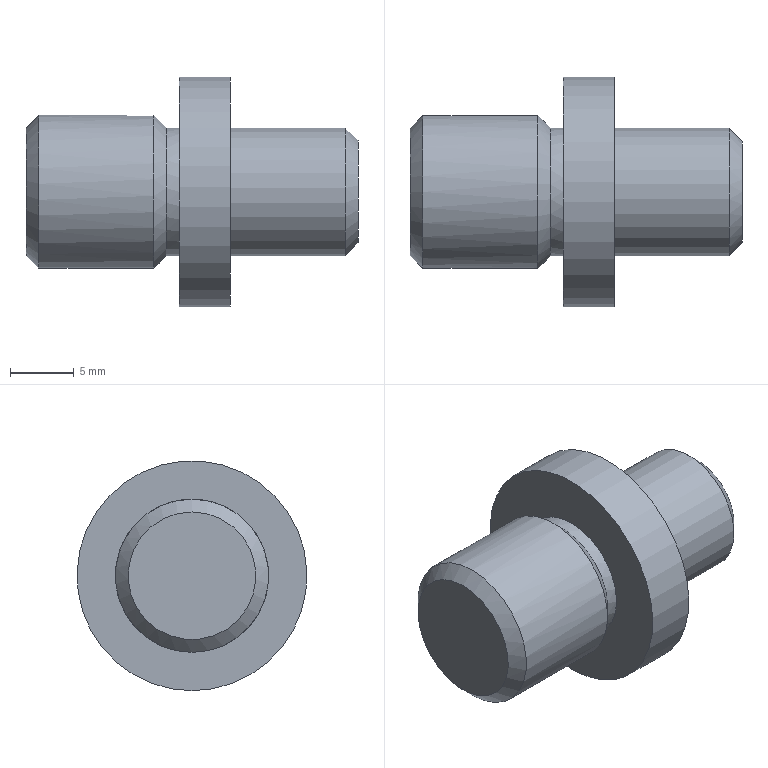Component | NX | A_LOCATING_PIN | 1 solid | 11 faces | box 26 x 18 x 18 mm | volume 3076 mm3 | plane 4 | cylinder 4 | cone 3 | commonest cylinder face diameters 10 x2 12 x1 18 x1
STEP:
#1=CARTESIAN_POINT('',(0.,0.,0.));
#2=DIRECTION('',(0.,0.,1.));
#3=DIRECTION('',(1.,0.,0.));
#4=AXIS2_PLACEMENT_3D('',#1,#2,#3);
#5=CARTESIAN_POINT('',(-41.,13.9,-11.5));
#6=VERTEX_POINT('',#5);
#7=CARTESIAN_POINT('',(-41.,13.9,-16.5));
#8=DIRECTION('',(-1.,0.,0.));
#9=DIRECTION('',(0.,0.,1.));
#10=AXIS2_PLACEMENT_3D('',#7,#8,#9);
#11=CIRCLE('',#10,5.);
#12=CARTESIAN_POINT('',(-41.,13.9,-16.5));
#13=DIRECTION('',(-1.,0.,0.));
#14=DIRECTION('',(0.,0.,1.));
#15=AXIS2_PLACEMENT_3D('',#12,#13,#14);
#16=PLANE('',#15);
#17=CARTESIAN_POINT('',(0.,0.));
#18=DIRECTION('',(1.,0.));
#19=AXIS2_PLACEMENT_2D('',#17,#18);
#20=CIRCLE('',#19,5.);
#21=(GEOMETRIC_REPRESENTATION_CONTEXT(2)PARAMETRIC_REPRESENTATION_CONTEXT()REPRESENTATION_CONTEXT('',''));
#22=DEFINITIONAL_REPRESENTATION('',(#20),#21);
#23=PCURVE('',#16,#22);
#24=CARTESIAN_POINT('',(-40.,13.9,-16.5));
#25=DIRECTION('',(1.,0.,0.));
#26=DIRECTION('',(0.,0.,-1.));
#27=AXIS2_PLACEMENT_3D('',#24,#25,#26);
#28=CONICAL_SURFACE('',#27,6.,0.7854);
#29=CARTESIAN_POINT('',(9.425,-1.));
#30=DIRECTION('',(-1.,0.));
#31=VECTOR('',#30,1.);
#32=LINE('',#29,#31);
#33=(GEOMETRIC_REPRESENTATION_CONTEXT(2)PARAMETRIC_REPRESENTATION_CONTEXT()REPRESENTATION_CONTEXT('',''));
#34=DEFINITIONAL_REPRESENTATION('',(#32),#33);
#35=PCURVE('',#28,#34);
#36=SURFACE_CURVE('',#11,(#23,#35),.PCURVE_S1.);
#37=EDGE_CURVE('',#6,#6,#36,.T.);
#38=ORIENTED_EDGE('',*,*,#37,.T.);
#39=EDGE_LOOP('',(#38));
#40=FACE_BOUND('',#39,.T.);
#41=ADVANCED_FACE('',(#40),#16,.T.);
#42=CARTESIAN_POINT('',(-31.,13.9,-22.5));
#43=VERTEX_POINT('',#42);
#44=CARTESIAN_POINT('',(-31.,13.9,-16.5));
#45=DIRECTION('',(-1.,0.,0.));
#46=DIRECTION('',(0.,0.,-1.));
#47=AXIS2_PLACEMENT_3D('',#44,#45,#46);
#48=CIRCLE('',#47,6.);
#49=CARTESIAN_POINT('',(-41.,13.9,-16.5));
#50=DIRECTION('',(1.,0.,0.));
#51=DIRECTION('',(0.,0.,-1.));
#52=AXIS2_PLACEMENT_3D('',#49,#50,#51);
#53=CYLINDRICAL_SURFACE('',#52,6.);
#54=CARTESIAN_POINT('',(6.283,10.));
#55=DIRECTION('',(-1.,0.));
#56=VECTOR('',#55,1.);
#57=LINE('',#54,#56);
#58=(GEOMETRIC_REPRESENTATION_CONTEXT(2)PARAMETRIC_REPRESENTATION_CONTEXT()REPRESENTATION_CONTEXT('',''));
#59=DEFINITIONAL_REPRESENTATION('',(#57),#58);
#60=PCURVE('',#53,#59);
#61=CARTESIAN_POINT('',(-31.,13.9,-16.5));
#62=DIRECTION('',(-1.,0.,0.));
#63=DIRECTION('',(0.,0.,1.));
#64=AXIS2_PLACEMENT_3D('',#61,#62,#63);
#65=CONICAL_SURFACE('',#64,6.,0.7854);
#66=CARTESIAN_POINT('',(3.142,0.));
#67=DIRECTION('',(1.,0.));
#68=VECTOR('',#67,1.);
#69=LINE('',#66,#68);
#70=(GEOMETRIC_REPRESENTATION_CONTEXT(2)PARAMETRIC_REPRESENTATION_CONTEXT()REPRESENTATION_CONTEXT('',''));
#71=DEFINITIONAL_REPRESENTATION('',(#69),#70);
#72=PCURVE('',#65,#71);
#73=SURFACE_CURVE('',#48,(#60,#72),.PCURVE_S1.);
#74=EDGE_CURVE('',#43,#43,#73,.T.);
#75=ORIENTED_EDGE('',*,*,#74,.T.);
#76=CARTESIAN_POINT('',(-40.,13.9,-22.5));
#77=VERTEX_POINT('',#76);
#78=CARTESIAN_POINT('',(-40.,13.9,-22.5));
#79=CARTESIAN_POINT('',(-31.,13.9,-22.5));
#80=B_SPLINE_CURVE_WITH_KNOTS('',1,(#78,#79),.UNSPECIFIED.,.F.,.F.,(2,2),(1.,10.),.PIECEWISE_BEZIER_KNOTS.);
#81=CARTESIAN_POINT('',(0.,0.));
#82=DIRECTION('',(0.,1.));
#83=VECTOR('',#82,1.);
#84=LINE('',#81,#83);
#85=(GEOMETRIC_REPRESENTATION_CONTEXT(2)PARAMETRIC_REPRESENTATION_CONTEXT()REPRESENTATION_CONTEXT('',''));
#86=DEFINITIONAL_REPRESENTATION('',(#84),#85);
#87=PCURVE('',#53,#86);
#88=CARTESIAN_POINT('',(6.283,0.));
#89=DIRECTION('',(0.,1.));
#90=VECTOR('',#89,1.);
#91=LINE('',#88,#90);
#92=(GEOMETRIC_REPRESENTATION_CONTEXT(2)PARAMETRIC_REPRESENTATION_CONTEXT()REPRESENTATION_CONTEXT('',''));
#93=DEFINITIONAL_REPRESENTATION('',(#91),#92);
#94=PCURVE('',#53,#93);
#95=SEAM_CURVE('',#80,(#87,#94),.PCURVE_S1.);
#96=EDGE_CURVE('',#77,#43,#95,.T.);
#97=ORIENTED_EDGE('',*,*,#96,.F.);
#98=CARTESIAN_POINT('',(-40.,13.9,-10.5));
#99=VERTEX_POINT('',#98);
#100=CARTESIAN_POINT('',(-40.,13.9,-16.5));
#101=DIRECTION('',(1.,0.,0.));
#102=DIRECTION('',(0.,0.,1.));
#103=AXIS2_PLACEMENT_3D('',#100,#101,#102);
#104=CIRCLE('',#103,6.);
#105=CARTESIAN_POINT('',(-3.142,1.));
#106=DIRECTION('',(1.,0.));
#107=VECTOR('',#106,1.);
#108=LINE('',#105,#107);
#109=(GEOMETRIC_REPRESENTATION_CONTEXT(2)PARAMETRIC_REPRESENTATION_CONTEXT()REPRESENTATION_CONTEXT('',''));
#110=DEFINITIONAL_REPRESENTATION('',(#108),#109);
#111=PCURVE('',#53,#110);
#112=CARTESIAN_POINT('',(3.142,0.));
#113=DIRECTION('',(1.,0.));
#114=VECTOR('',#113,1.);
#115=LINE('',#112,#114);
#116=(GEOMETRIC_REPRESENTATION_CONTEXT(2)PARAMETRIC_REPRESENTATION_CONTEXT()REPRESENTATION_CONTEXT('',''));
#117=DEFINITIONAL_REPRESENTATION('',(#115),#116);
#118=PCURVE('',#28,#117);
#119=SURFACE_CURVE('',#104,(#111,#118),.PCURVE_S1.);
#120=EDGE_CURVE('',#77,#99,#119,.T.);
#121=ORIENTED_EDGE('',*,*,#120,.T.);
#122=CARTESIAN_POINT('',(-40.,13.9,-16.5));
#123=DIRECTION('',(1.,0.,0.));
#124=DIRECTION('',(0.,0.,1.));
#125=AXIS2_PLACEMENT_3D('',#122,#123,#124);
#126=CIRCLE('',#125,6.);
#127=CARTESIAN_POINT('',(3.142,1.));
#128=DIRECTION('',(1.,0.));
#129=VECTOR('',#128,1.);
#130=LINE('',#127,#129);
#131=(GEOMETRIC_REPRESENTATION_CONTEXT(2)PARAMETRIC_REPRESENTATION_CONTEXT()REPRESENTATION_CONTEXT('',''));
#132=DEFINITIONAL_REPRESENTATION('',(#130),#131);
#133=PCURVE('',#53,#132);
#134=CARTESIAN_POINT('',(3.142,0.));
#135=DIRECTION('',(1.,0.));
#136=VECTOR('',#135,1.);
#137=LINE('',#134,#136);
#138=(GEOMETRIC_REPRESENTATION_CONTEXT(2)PARAMETRIC_REPRESENTATION_CONTEXT()REPRESENTATION_CONTEXT('',''));
#139=DEFINITIONAL_REPRESENTATION('',(#137),#138);
#140=PCURVE('',#28,#139);
#141=SURFACE_CURVE('',#126,(#133,#140),.PCURVE_S1.);
#142=EDGE_CURVE('',#99,#77,#141,.T.);
#143=ORIENTED_EDGE('',*,*,#142,.T.);
#144=ORIENTED_EDGE('',*,*,#96,.T.);
#145=EDGE_LOOP('',(#75,#97,#121,#143,#144));
#146=FACE_BOUND('',#145,.T.);
#147=ADVANCED_FACE('',(#146),#53,.T.);
#148=CARTESIAN_POINT('',(-29.,13.9,-21.5));
#149=VERTEX_POINT('',#148);
#150=CARTESIAN_POINT('',(-29.,13.9,-11.5));
#151=VERTEX_POINT('',#150);
#152=CARTESIAN_POINT('',(-29.,13.9,-16.5));
#153=DIRECTION('',(1.,0.,0.));
#154=DIRECTION('',(0.,0.,1.));
#155=AXIS2_PLACEMENT_3D('',#152,#153,#154);
#156=CIRCLE('',#155,5.);
#157=CARTESIAN_POINT('',(-30.,13.9,-16.5));
#158=DIRECTION('',(1.,0.,0.));
#159=DIRECTION('',(0.,0.,-1.));
#160=AXIS2_PLACEMENT_3D('',#157,#158,#159);
#161=CYLINDRICAL_SURFACE('',#160,5.);
#162=CARTESIAN_POINT('',(-3.142,1.));
#163=DIRECTION('',(1.,0.));
#164=VECTOR('',#163,1.);
#165=LINE('',#162,#164);
#166=(GEOMETRIC_REPRESENTATION_CONTEXT(2)PARAMETRIC_REPRESENTATION_CONTEXT()REPRESENTATION_CONTEXT('',''));
#167=DEFINITIONAL_REPRESENTATION('',(#165),#166);
#168=PCURVE('',#161,#167);
#169=CARTESIAN_POINT('',(-29.,13.9,-16.5));
#170=DIRECTION('',(-1.,0.,0.));
#171=DIRECTION('',(0.,0.,1.));
#172=AXIS2_PLACEMENT_3D('',#169,#170,#171);
#173=PLANE('',#172);
#174=CARTESIAN_POINT('',(5.,0.));
#175=CARTESIAN_POINT('',(5.,-8.66));
#176=CARTESIAN_POINT('',(-2.5,-4.33));
#177=CARTESIAN_POINT('',(-10.,-0.));
#178=CARTESIAN_POINT('',(-2.5,4.33));
#179=CARTESIAN_POINT('',(5.,8.66));
#180=CARTESIAN_POINT('',(5.,0.));
#181=(BOUNDED_CURVE()B_SPLINE_CURVE(2,(#174,#175,#176,#177,#178,#179,#180),.UNSPECIFIED.,.T.,.F.)B_SPLINE_CURVE_WITH_KNOTS((1,2,2,2,2,1),(-2.094,0.,2.094,4.189,6.283,8.378),.UNSPECIFIED.)CURVE()GEOMETRIC_REPRESENTATION_ITEM()RATIONAL_B_SPLINE_CURVE((1.,0.5,1.,0.5,1.,0.5,1.))REPRESENTATION_ITEM(''));
#182=(GEOMETRIC_REPRESENTATION_CONTEXT(2)PARAMETRIC_REPRESENTATION_CONTEXT()REPRESENTATION_CONTEXT('',''));
#183=DEFINITIONAL_REPRESENTATION('',(#181),#182);
#184=PCURVE('',#173,#183);
#185=SURFACE_CURVE('',#156,(#168,#184),.PCURVE_S1.);
#186=EDGE_CURVE('',#149,#151,#185,.T.);
#187=ORIENTED_EDGE('',*,*,#186,.F.);
#188=CARTESIAN_POINT('',(-30.,13.9,-21.5));
#189=VERTEX_POINT('',#188);
#190=CARTESIAN_POINT('',(-30.,13.9,-21.5));
#191=CARTESIAN_POINT('',(-29.,13.9,-21.5));
#192=B_SPLINE_CURVE_WITH_KNOTS('',1,(#190,#191),.UNSPECIFIED.,.F.,.F.,(2,2),(0.,1.),.PIECEWISE_BEZIER_KNOTS.);
#193=CARTESIAN_POINT('',(0.,0.));
#194=DIRECTION('',(0.,1.));
#195=VECTOR('',#194,1.);
#196=LINE('',#193,#195);
#197=(GEOMETRIC_REPRESENTATION_CONTEXT(2)PARAMETRIC_REPRESENTATION_CONTEXT()REPRESENTATION_CONTEXT('',''));
#198=DEFINITIONAL_REPRESENTATION('',(#196),#197);
#199=PCURVE('',#161,#198);
#200=CARTESIAN_POINT('',(6.283,0.));
#201=DIRECTION('',(0.,1.));
#202=VECTOR('',#201,1.);
#203=LINE('',#200,#202);
#204=(GEOMETRIC_REPRESENTATION_CONTEXT(2)PARAMETRIC_REPRESENTATION_CONTEXT()REPRESENTATION_CONTEXT('',''));
#205=DEFINITIONAL_REPRESENTATION('',(#203),#204);
#206=PCURVE('',#161,#205);
#207=SEAM_CURVE('',#192,(#199,#206),.PCURVE_S1.);
#208=EDGE_CURVE('',#189,#149,#207,.T.);
#209=ORIENTED_EDGE('',*,*,#208,.F.);
#210=CARTESIAN_POINT('',(-30.,13.9,-16.5));
#211=DIRECTION('',(1.,0.,0.));
#212=DIRECTION('',(0.,0.,-1.));
#213=AXIS2_PLACEMENT_3D('',#210,#211,#212);
#214=CIRCLE('',#213,5.);
#215=CARTESIAN_POINT('',(0.,0.));
#216=DIRECTION('',(1.,0.));
#217=VECTOR('',#216,1.);
#218=LINE('',#215,#217);
#219=(GEOMETRIC_REPRESENTATION_CONTEXT(2)PARAMETRIC_REPRESENTATION_CONTEXT()REPRESENTATION_CONTEXT('',''));
#220=DEFINITIONAL_REPRESENTATION('',(#218),#219);
#221=PCURVE('',#161,#220);
#222=CARTESIAN_POINT('',(9.425,-1.));
#223=DIRECTION('',(-1.,0.));
#224=VECTOR('',#223,1.);
#225=LINE('',#222,#224);
#226=(GEOMETRIC_REPRESENTATION_CONTEXT(2)PARAMETRIC_REPRESENTATION_CONTEXT()REPRESENTATION_CONTEXT('',''));
#227=DEFINITIONAL_REPRESENTATION('',(#225),#226);
#228=PCURVE('',#65,#227);
#229=SURFACE_CURVE('',#214,(#221,#228),.PCURVE_S1.);
#230=EDGE_CURVE('',#189,#189,#229,.T.);
#231=ORIENTED_EDGE('',*,*,#230,.T.);
#232=ORIENTED_EDGE('',*,*,#208,.T.);
#233=CARTESIAN_POINT('',(-29.,13.9,-16.5));
#234=DIRECTION('',(1.,0.,0.));
#235=DIRECTION('',(0.,0.,1.));
#236=AXIS2_PLACEMENT_3D('',#233,#234,#235);
#237=CIRCLE('',#236,5.);
#238=CARTESIAN_POINT('',(3.142,1.));
#239=DIRECTION('',(1.,0.));
#240=VECTOR('',#239,1.);
#241=LINE('',#238,#240);
#242=(GEOMETRIC_REPRESENTATION_CONTEXT(2)PARAMETRIC_REPRESENTATION_CONTEXT()REPRESENTATION_CONTEXT('',''));
#243=DEFINITIONAL_REPRESENTATION('',(#241),#242);
#244=PCURVE('',#161,#243);
#245=CARTESIAN_POINT('',(5.,0.));
#246=CARTESIAN_POINT('',(5.,-8.66));
#247=CARTESIAN_POINT('',(-2.5,-4.33));
#248=CARTESIAN_POINT('',(-10.,-0.));
#249=CARTESIAN_POINT('',(-2.5,4.33));
#250=CARTESIAN_POINT('',(5.,8.66));
#251=CARTESIAN_POINT('',(5.,0.));
#252=(BOUNDED_CURVE()B_SPLINE_CURVE(2,(#245,#246,#247,#248,#249,#250,#251),.UNSPECIFIED.,.T.,.F.)B_SPLINE_CURVE_WITH_KNOTS((1,2,2,2,2,1),(-2.094,0.,2.094,4.189,6.283,8.378),.UNSPECIFIED.)CURVE()GEOMETRIC_REPRESENTATION_ITEM()RATIONAL_B_SPLINE_CURVE((1.,0.5,1.,0.5,1.,0.5,1.))REPRESENTATION_ITEM(''));
#253=(GEOMETRIC_REPRESENTATION_CONTEXT(2)PARAMETRIC_REPRESENTATION_CONTEXT()REPRESENTATION_CONTEXT('',''));
#254=DEFINITIONAL_REPRESENTATION('',(#252),#253);
#255=PCURVE('',#173,#254);
#256=SURFACE_CURVE('',#237,(#244,#255),.PCURVE_S1.);
#257=EDGE_CURVE('',#151,#149,#256,.T.);
#258=ORIENTED_EDGE('',*,*,#257,.F.);
#259=EDGE_LOOP('',(#187,#209,#231,#232,#258));
#260=FACE_BOUND('',#259,.T.);
#261=ADVANCED_FACE('',(#260),#161,.T.);
#262=CARTESIAN_POINT('',(-25.,13.9,-21.5));
#263=VERTEX_POINT('',#262);
#264=CARTESIAN_POINT('',(-25.,13.9,-16.5));
#265=DIRECTION('',(1.,0.,0.));
#266=DIRECTION('',(0.,0.,-1.));
#267=AXIS2_PLACEMENT_3D('',#264,#265,#266);
#268=CIRCLE('',#267,5.);
#269=CARTESIAN_POINT('',(-25.,13.9,-16.5));
#270=DIRECTION('',(1.,0.,0.));
#271=DIRECTION('',(0.,0.,-1.));
#272=AXIS2_PLACEMENT_3D('',#269,#270,#271);
#273=PLANE('',#272);
#274=CARTESIAN_POINT('',(0.,0.));
#275=DIRECTION('',(1.,0.));
#276=AXIS2_PLACEMENT_2D('',#274,#275);
#277=CIRCLE('',#276,5.);
#278=(GEOMETRIC_REPRESENTATION_CONTEXT(2)PARAMETRIC_REPRESENTATION_CONTEXT()REPRESENTATION_CONTEXT('',''));
#279=DEFINITIONAL_REPRESENTATION('',(#277),#278);
#280=PCURVE('',#273,#279);
#281=CARTESIAN_POINT('',(-25.,13.9,-16.5));
#282=DIRECTION('',(1.,0.,0.));
#283=DIRECTION('',(0.,0.,-1.));
#284=AXIS2_PLACEMENT_3D('',#281,#282,#283);
#285=CYLINDRICAL_SURFACE('',#284,5.);
#286=CARTESIAN_POINT('',(0.,0.));
#287=DIRECTION('',(1.,0.));
#288=VECTOR('',#287,1.);
#289=LINE('',#286,#288);
#290=(GEOMETRIC_REPRESENTATION_CONTEXT(2)PARAMETRIC_REPRESENTATION_CONTEXT()REPRESENTATION_CONTEXT('',''));
#291=DEFINITIONAL_REPRESENTATION('',(#289),#290);
#292=PCURVE('',#285,#291);
#293=SURFACE_CURVE('',#268,(#280,#292),.PCURVE_S1.);
#294=EDGE_CURVE('',#263,#263,#293,.T.);
#295=ORIENTED_EDGE('',*,*,#294,.F.);
#296=EDGE_LOOP('',(#295));
#297=FACE_BOUND('',#296,.T.);
#298=CARTESIAN_POINT('',(-25.,13.9,-25.5));
#299=VERTEX_POINT('',#298);
#300=CARTESIAN_POINT('',(-25.,13.9,-16.5));
#301=DIRECTION('',(-1.,0.,0.));
#302=DIRECTION('',(0.,0.,-1.));
#303=AXIS2_PLACEMENT_3D('',#300,#301,#302);
#304=CIRCLE('',#303,9.);
#305=CARTESIAN_POINT('',(9.,0.));
#306=CARTESIAN_POINT('',(9.,-15.588));
#307=CARTESIAN_POINT('',(-4.5,-7.794));
#308=CARTESIAN_POINT('',(-18.,-0.));
#309=CARTESIAN_POINT('',(-4.5,7.794));
#310=CARTESIAN_POINT('',(9.,15.588));
#311=CARTESIAN_POINT('',(9.,0.));
#312=(BOUNDED_CURVE()B_SPLINE_CURVE(2,(#305,#306,#307,#308,#309,#310,#311),.UNSPECIFIED.,.T.,.F.)B_SPLINE_CURVE_WITH_KNOTS((1,2,2,2,2,1),(-2.094,0.,2.094,4.189,6.283,8.378),.UNSPECIFIED.)CURVE()GEOMETRIC_REPRESENTATION_ITEM()RATIONAL_B_SPLINE_CURVE((1.,0.5,1.,0.5,1.,0.5,1.))REPRESENTATION_ITEM(''));
#313=(GEOMETRIC_REPRESENTATION_CONTEXT(2)PARAMETRIC_REPRESENTATION_CONTEXT()REPRESENTATION_CONTEXT('',''));
#314=DEFINITIONAL_REPRESENTATION('',(#312),#313);
#315=PCURVE('',#273,#314);
#316=CARTESIAN_POINT('',(-29.,13.9,-16.5));
#317=DIRECTION('',(1.,0.,0.));
#318=DIRECTION('',(0.,0.,-1.));
#319=AXIS2_PLACEMENT_3D('',#316,#317,#318);
#320=CYLINDRICAL_SURFACE('',#319,9.);
#321=CARTESIAN_POINT('',(6.283,4.));
#322=DIRECTION('',(-1.,0.));
#323=VECTOR('',#322,1.);
#324=LINE('',#321,#323);
#325=(GEOMETRIC_REPRESENTATION_CONTEXT(2)PARAMETRIC_REPRESENTATION_CONTEXT()REPRESENTATION_CONTEXT('',''));
#326=DEFINITIONAL_REPRESENTATION('',(#324),#325);
#327=PCURVE('',#320,#326);
#328=SURFACE_CURVE('',#304,(#315,#327),.PCURVE_S1.);
#329=EDGE_CURVE('',#299,#299,#328,.T.);
#330=ORIENTED_EDGE('',*,*,#329,.F.);
#331=EDGE_LOOP('',(#330));
#332=FACE_BOUND('',#331,.T.);
#333=ADVANCED_FACE('',(#297,#332),#273,.T.);
#334=ORIENTED_EDGE('',*,*,#257,.T.);
#335=ORIENTED_EDGE('',*,*,#186,.T.);
#336=EDGE_LOOP('',(#334,#335));
#337=FACE_BOUND('',#336,.T.);
#338=CARTESIAN_POINT('',(-29.,13.9,-25.5));
#339=VERTEX_POINT('',#338);
#340=CARTESIAN_POINT('',(-29.,13.9,-16.5));
#341=DIRECTION('',(1.,0.,0.));
#342=DIRECTION('',(0.,0.,-1.));
#343=AXIS2_PLACEMENT_3D('',#340,#341,#342);
#344=CIRCLE('',#343,9.);
#345=CARTESIAN_POINT('',(-9.,0.));
#346=CARTESIAN_POINT('',(-9.,15.588));
#347=CARTESIAN_POINT('',(4.5,7.794));
#348=CARTESIAN_POINT('',(18.,0.));
#349=CARTESIAN_POINT('',(4.5,-7.794));
#350=CARTESIAN_POINT('',(-9.,-15.588));
#351=CARTESIAN_POINT('',(-9.,0.));
#352=(BOUNDED_CURVE()B_SPLINE_CURVE(2,(#345,#346,#347,#348,#349,#350,#351),.UNSPECIFIED.,.T.,.F.)B_SPLINE_CURVE_WITH_KNOTS((1,2,2,2,2,1),(-2.094,0.,2.094,4.189,6.283,8.378),.UNSPECIFIED.)CURVE()GEOMETRIC_REPRESENTATION_ITEM()RATIONAL_B_SPLINE_CURVE((1.,0.5,1.,0.5,1.,0.5,1.))REPRESENTATION_ITEM(''));
#353=(GEOMETRIC_REPRESENTATION_CONTEXT(2)PARAMETRIC_REPRESENTATION_CONTEXT()REPRESENTATION_CONTEXT('',''));
#354=DEFINITIONAL_REPRESENTATION('',(#352),#353);
#355=PCURVE('',#173,#354);
#356=CARTESIAN_POINT('',(0.,0.));
#357=DIRECTION('',(1.,0.));
#358=VECTOR('',#357,1.);
#359=LINE('',#356,#358);
#360=(GEOMETRIC_REPRESENTATION_CONTEXT(2)PARAMETRIC_REPRESENTATION_CONTEXT()REPRESENTATION_CONTEXT('',''));
#361=DEFINITIONAL_REPRESENTATION('',(#359),#360);
#362=PCURVE('',#320,#361);
#363=SURFACE_CURVE('',#344,(#355,#362),.PCURVE_S1.);
#364=EDGE_CURVE('',#339,#339,#363,.T.);
#365=ORIENTED_EDGE('',*,*,#364,.F.);
#366=EDGE_LOOP('',(#365));
#367=FACE_BOUND('',#366,.T.);
#368=ADVANCED_FACE('',(#337,#367),#173,.T.);
#369=ORIENTED_EDGE('',*,*,#329,.T.);
#370=CARTESIAN_POINT('',(-29.,13.9,-25.5));
#371=CARTESIAN_POINT('',(-25.,13.9,-25.5));
#372=B_SPLINE_CURVE_WITH_KNOTS('',1,(#370,#371),.UNSPECIFIED.,.F.,.F.,(2,2),(0.,4.),.PIECEWISE_BEZIER_KNOTS.);
#373=CARTESIAN_POINT('',(0.,0.));
#374=DIRECTION('',(0.,1.));
#375=VECTOR('',#374,1.);
#376=LINE('',#373,#375);
#377=(GEOMETRIC_REPRESENTATION_CONTEXT(2)PARAMETRIC_REPRESENTATION_CONTEXT()REPRESENTATION_CONTEXT('',''));
#378=DEFINITIONAL_REPRESENTATION('',(#376),#377);
#379=PCURVE('',#320,#378);
#380=CARTESIAN_POINT('',(6.283,0.));
#381=DIRECTION('',(0.,1.));
#382=VECTOR('',#381,1.);
#383=LINE('',#380,#382);
#384=(GEOMETRIC_REPRESENTATION_CONTEXT(2)PARAMETRIC_REPRESENTATION_CONTEXT()REPRESENTATION_CONTEXT('',''));
#385=DEFINITIONAL_REPRESENTATION('',(#383),#384);
#386=PCURVE('',#320,#385);
#387=SEAM_CURVE('',#372,(#379,#386),.PCURVE_S1.);
#388=EDGE_CURVE('',#339,#299,#387,.T.);
#389=ORIENTED_EDGE('',*,*,#388,.F.);
#390=ORIENTED_EDGE('',*,*,#364,.T.);
#391=ORIENTED_EDGE('',*,*,#388,.T.);
#392=EDGE_LOOP('',(#369,#389,#390,#391));
#393=FACE_BOUND('',#392,.T.);
#394=ADVANCED_FACE('',(#393),#320,.T.);
#395=CARTESIAN_POINT('',(-16.,13.9,-21.5));
#396=VERTEX_POINT('',#395);
#397=CARTESIAN_POINT('',(-16.,13.9,-16.5));
#398=DIRECTION('',(-1.,0.,0.));
#399=DIRECTION('',(0.,0.,-1.));
#400=AXIS2_PLACEMENT_3D('',#397,#398,#399);
#401=CIRCLE('',#400,5.);
#402=CARTESIAN_POINT('',(6.283,9.));
#403=DIRECTION('',(-1.,0.));
#404=VECTOR('',#403,1.);
#405=LINE('',#402,#404);
#406=(GEOMETRIC_REPRESENTATION_CONTEXT(2)PARAMETRIC_REPRESENTATION_CONTEXT()REPRESENTATION_CONTEXT('',''));
#407=DEFINITIONAL_REPRESENTATION('',(#405),#406);
#408=PCURVE('',#285,#407);
#409=CARTESIAN_POINT('',(-16.,13.9,-16.5));
#410=DIRECTION('',(-1.,0.,0.));
#411=DIRECTION('',(0.,0.,1.));
#412=AXIS2_PLACEMENT_3D('',#409,#410,#411);
#413=CONICAL_SURFACE('',#412,5.,0.7854);
#414=CARTESIAN_POINT('',(3.142,0.));
#415=DIRECTION('',(1.,0.));
#416=VECTOR('',#415,1.);
#417=LINE('',#414,#416);
#418=(GEOMETRIC_REPRESENTATION_CONTEXT(2)PARAMETRIC_REPRESENTATION_CONTEXT()REPRESENTATION_CONTEXT('',''));
#419=DEFINITIONAL_REPRESENTATION('',(#417),#418);
#420=PCURVE('',#413,#419);
#421=SURFACE_CURVE('',#401,(#408,#420),.PCURVE_S1.);
#422=EDGE_CURVE('',#396,#396,#421,.T.);
#423=ORIENTED_EDGE('',*,*,#422,.T.);
#424=CARTESIAN_POINT('',(-25.,13.9,-21.5));
#425=CARTESIAN_POINT('',(-16.,13.9,-21.5));
#426=B_SPLINE_CURVE_WITH_KNOTS('',1,(#424,#425),.UNSPECIFIED.,.F.,.F.,(2,2),(0.,9.),.PIECEWISE_BEZIER_KNOTS.);
#427=CARTESIAN_POINT('',(0.,0.));
#428=DIRECTION('',(0.,1.));
#429=VECTOR('',#428,1.);
#430=LINE('',#427,#429);
#431=(GEOMETRIC_REPRESENTATION_CONTEXT(2)PARAMETRIC_REPRESENTATION_CONTEXT()REPRESENTATION_CONTEXT('',''));
#432=DEFINITIONAL_REPRESENTATION('',(#430),#431);
#433=PCURVE('',#285,#432);
#434=CARTESIAN_POINT('',(6.283,0.));
#435=DIRECTION('',(0.,1.));
#436=VECTOR('',#435,1.);
#437=LINE('',#434,#436);
#438=(GEOMETRIC_REPRESENTATION_CONTEXT(2)PARAMETRIC_REPRESENTATION_CONTEXT()REPRESENTATION_CONTEXT('',''));
#439=DEFINITIONAL_REPRESENTATION('',(#437),#438);
#440=PCURVE('',#285,#439);
#441=SEAM_CURVE('',#426,(#433,#440),.PCURVE_S1.);
#442=EDGE_CURVE('',#263,#396,#441,.T.);
#443=ORIENTED_EDGE('',*,*,#442,.F.);
#444=ORIENTED_EDGE('',*,*,#294,.T.);
#445=ORIENTED_EDGE('',*,*,#442,.T.);
#446=EDGE_LOOP('',(#423,#443,#444,#445));
#447=FACE_BOUND('',#446,.T.);
#448=ADVANCED_FACE('',(#447),#285,.T.);
#449=CARTESIAN_POINT('',(-15.,13.9,-20.5));
#450=VERTEX_POINT('',#449);
#451=CARTESIAN_POINT('',(-15.,13.9,-16.5));
#452=DIRECTION('',(1.,0.,0.));
#453=DIRECTION('',(0.,0.,-1.));
#454=AXIS2_PLACEMENT_3D('',#451,#452,#453);
#455=CIRCLE('',#454,4.);
#456=CARTESIAN_POINT('',(-15.,13.9,-16.5));
#457=DIRECTION('',(1.,0.,0.));
#458=DIRECTION('',(0.,0.,-1.));
#459=AXIS2_PLACEMENT_3D('',#456,#457,#458);
#460=PLANE('',#459);
#461=CARTESIAN_POINT('',(0.,0.));
#462=DIRECTION('',(1.,0.));
#463=AXIS2_PLACEMENT_2D('',#461,#462);
#464=CIRCLE('',#463,4.);
#465=(GEOMETRIC_REPRESENTATION_CONTEXT(2)PARAMETRIC_REPRESENTATION_CONTEXT()REPRESENTATION_CONTEXT('',''));
#466=DEFINITIONAL_REPRESENTATION('',(#464),#465);
#467=PCURVE('',#460,#466);
#468=CARTESIAN_POINT('',(9.425,-1.));
#469=DIRECTION('',(-1.,0.));
#470=VECTOR('',#469,1.);
#471=LINE('',#468,#470);
#472=(GEOMETRIC_REPRESENTATION_CONTEXT(2)PARAMETRIC_REPRESENTATION_CONTEXT()REPRESENTATION_CONTEXT('',''));
#473=DEFINITIONAL_REPRESENTATION('',(#471),#472);
#474=PCURVE('',#413,#473);
#475=SURFACE_CURVE('',#455,(#467,#474),.PCURVE_S1.);
#476=EDGE_CURVE('',#450,#450,#475,.T.);
#477=ORIENTED_EDGE('',*,*,#476,.T.);
#478=EDGE_LOOP('',(#477));
#479=FACE_BOUND('',#478,.T.);
#480=ADVANCED_FACE('',(#479),#460,.T.);
#481=ORIENTED_EDGE('',*,*,#476,.F.);
#482=CARTESIAN_POINT('',(-15.,13.9,-20.5));
#483=CARTESIAN_POINT('',(-16.,13.9,-21.5));
#484=B_SPLINE_CURVE_WITH_KNOTS('',1,(#482,#483),.UNSPECIFIED.,.F.,.F.,(2,2),(-1.414,0.),.PIECEWISE_BEZIER_KNOTS.);
#485=CARTESIAN_POINT('',(9.425,0.));
#486=DIRECTION('',(0.,1.));
#487=VECTOR('',#486,1.);
#488=LINE('',#485,#487);
#489=(GEOMETRIC_REPRESENTATION_CONTEXT(2)PARAMETRIC_REPRESENTATION_CONTEXT()REPRESENTATION_CONTEXT('',''));
#490=DEFINITIONAL_REPRESENTATION('',(#488),#489);
#491=PCURVE('',#413,#490);
#492=CARTESIAN_POINT('',(3.142,0.));
#493=DIRECTION('',(0.,1.));
#494=VECTOR('',#493,1.);
#495=LINE('',#492,#494);
#496=(GEOMETRIC_REPRESENTATION_CONTEXT(2)PARAMETRIC_REPRESENTATION_CONTEXT()REPRESENTATION_CONTEXT('',''));
#497=DEFINITIONAL_REPRESENTATION('',(#495),#496);
#498=PCURVE('',#413,#497);
#499=SEAM_CURVE('',#484,(#491,#498),.PCURVE_S1.);
#500=EDGE_CURVE('',#450,#396,#499,.T.);
#501=ORIENTED_EDGE('',*,*,#500,.T.);
#502=ORIENTED_EDGE('',*,*,#422,.F.);
#503=ORIENTED_EDGE('',*,*,#500,.F.);
#504=EDGE_LOOP('',(#481,#501,#502,#503));
#505=FACE_BOUND('',#504,.T.);
#506=ADVANCED_FACE('',(#505),#413,.T.);
#507=ORIENTED_EDGE('',*,*,#230,.F.);
#508=CARTESIAN_POINT('',(-30.,13.9,-21.5));
#509=CARTESIAN_POINT('',(-31.,13.9,-22.5));
#510=B_SPLINE_CURVE_WITH_KNOTS('',1,(#508,#509),.UNSPECIFIED.,.F.,.F.,(2,2),(-1.414,0.),.PIECEWISE_BEZIER_KNOTS.);
#511=CARTESIAN_POINT('',(9.425,0.));
#512=DIRECTION('',(0.,1.));
#513=VECTOR('',#512,1.);
#514=LINE('',#511,#513);
#515=(GEOMETRIC_REPRESENTATION_CONTEXT(2)PARAMETRIC_REPRESENTATION_CONTEXT()REPRESENTATION_CONTEXT('',''));
#516=DEFINITIONAL_REPRESENTATION('',(#514),#515);
#517=PCURVE('',#65,#516);
#518=CARTESIAN_POINT('',(3.142,0.));
#519=DIRECTION('',(0.,1.));
#520=VECTOR('',#519,1.);
#521=LINE('',#518,#520);
#522=(GEOMETRIC_REPRESENTATION_CONTEXT(2)PARAMETRIC_REPRESENTATION_CONTEXT()REPRESENTATION_CONTEXT('',''));
#523=DEFINITIONAL_REPRESENTATION('',(#521),#522);
#524=PCURVE('',#65,#523);
#525=SEAM_CURVE('',#510,(#517,#524),.PCURVE_S1.);
#526=EDGE_CURVE('',#189,#43,#525,.T.);
#527=ORIENTED_EDGE('',*,*,#526,.T.);
#528=ORIENTED_EDGE('',*,*,#74,.F.);
#529=ORIENTED_EDGE('',*,*,#526,.F.);
#530=EDGE_LOOP('',(#507,#527,#528,#529));
#531=FACE_BOUND('',#530,.T.);
#532=ADVANCED_FACE('',(#531),#65,.T.);
#533=ORIENTED_EDGE('',*,*,#37,.F.);
#534=CARTESIAN_POINT('',(-41.,13.9,-11.5));
#535=CARTESIAN_POINT('',(-40.,13.9,-10.5));
#536=B_SPLINE_CURVE_WITH_KNOTS('',1,(#534,#535),.UNSPECIFIED.,.F.,.F.,(2,2),(-1.414,0.),.PIECEWISE_BEZIER_KNOTS.);
#537=CARTESIAN_POINT('',(9.425,0.));
#538=DIRECTION('',(0.,1.));
#539=VECTOR('',#538,1.);
#540=LINE('',#537,#539);
#541=(GEOMETRIC_REPRESENTATION_CONTEXT(2)PARAMETRIC_REPRESENTATION_CONTEXT()REPRESENTATION_CONTEXT('',''));
#542=DEFINITIONAL_REPRESENTATION('',(#540),#541);
#543=PCURVE('',#28,#542);
#544=CARTESIAN_POINT('',(3.142,0.));
#545=DIRECTION('',(0.,1.));
#546=VECTOR('',#545,1.);
#547=LINE('',#544,#546);
#548=(GEOMETRIC_REPRESENTATION_CONTEXT(2)PARAMETRIC_REPRESENTATION_CONTEXT()REPRESENTATION_CONTEXT('',''));
#549=DEFINITIONAL_REPRESENTATION('',(#547),#548);
#550=PCURVE('',#28,#549);
#551=SEAM_CURVE('',#536,(#543,#550),.PCURVE_S1.);
#552=EDGE_CURVE('',#6,#99,#551,.T.);
#553=ORIENTED_EDGE('',*,*,#552,.T.);
#554=ORIENTED_EDGE('',*,*,#120,.F.);
#555=ORIENTED_EDGE('',*,*,#142,.F.);
#556=ORIENTED_EDGE('',*,*,#552,.F.);
#557=EDGE_LOOP('',(#533,#553,#554,#555,#556));
#558=FACE_BOUND('',#557,.T.);
#559=ADVANCED_FACE('',(#558),#28,.T.);
#560=CLOSED_SHELL('',(#41,#147,#261,#333,#368,#394,#448,#480,#506,#532,#559));
#561=MANIFOLD_SOLID_BREP('',#560);
#562=(LENGTH_UNIT()NAMED_UNIT(*)SI_UNIT(.MILLI.,.METRE.));
#563=UNCERTAINTY_MEASURE_WITH_UNIT(LENGTH_MEASURE(0.00001),#562,'','');
#564=(NAMED_UNIT(*)PLANE_ANGLE_UNIT()SI_UNIT($,.RADIAN.));
#565=(NAMED_UNIT(*)SI_UNIT($,.STERADIAN.)SOLID_ANGLE_UNIT());
#566=(GEOMETRIC_REPRESENTATION_CONTEXT(3)GLOBAL_UNCERTAINTY_ASSIGNED_CONTEXT((#563))GLOBAL_UNIT_ASSIGNED_CONTEXT((#562,#564,#565))REPRESENTATION_CONTEXT('',''));
#567=ADVANCED_BREP_SHAPE_REPRESENTATION('',(#4,#561),#566);